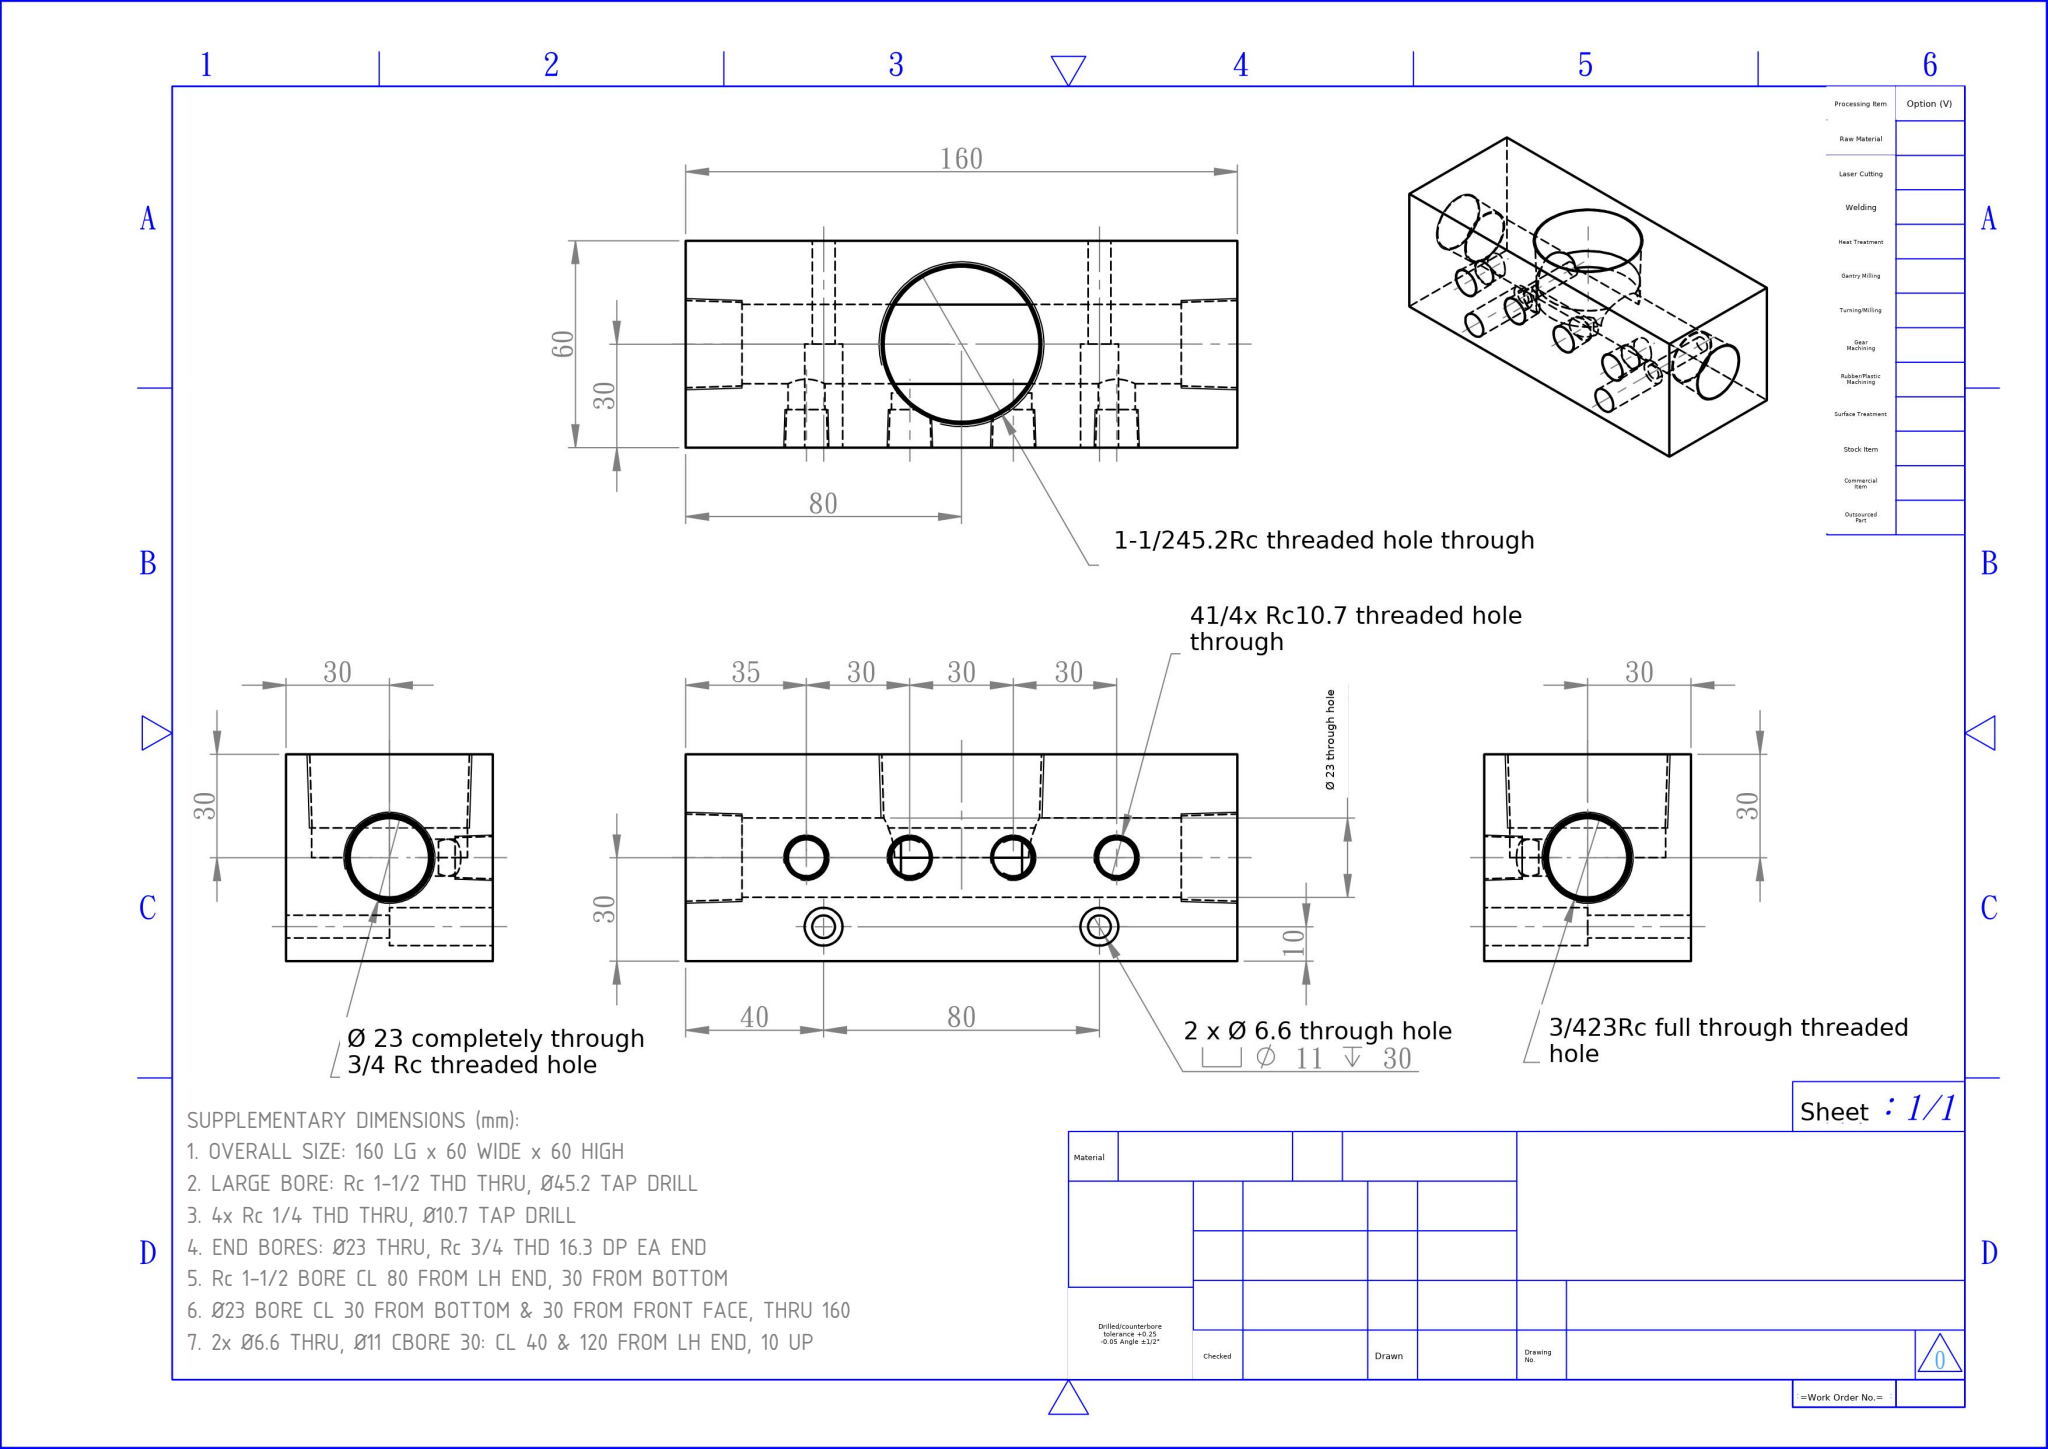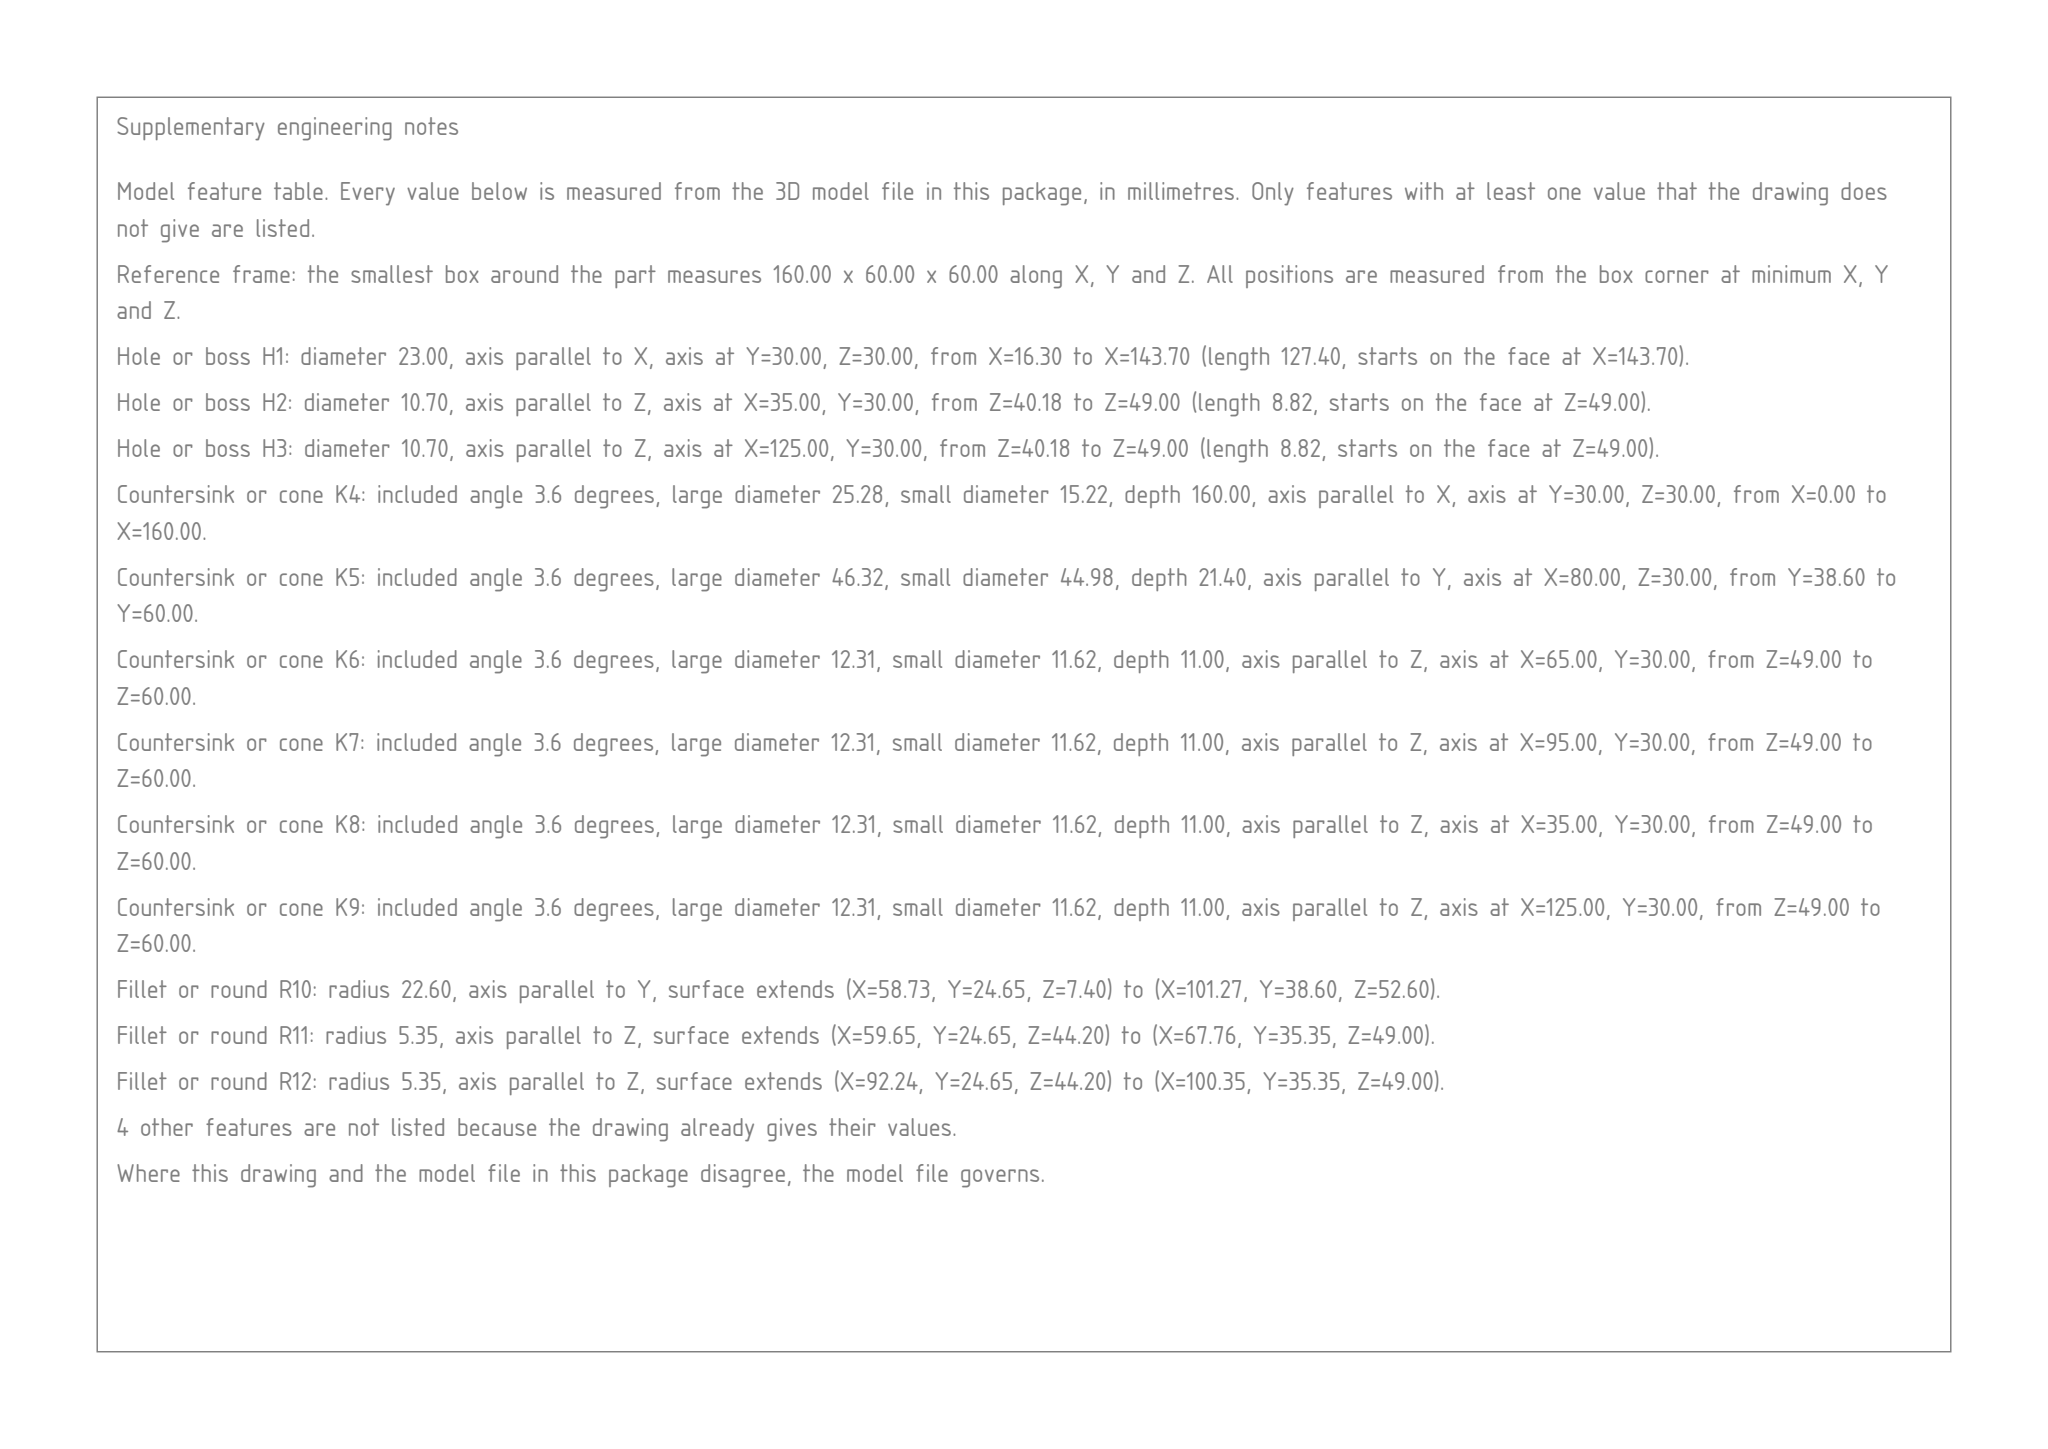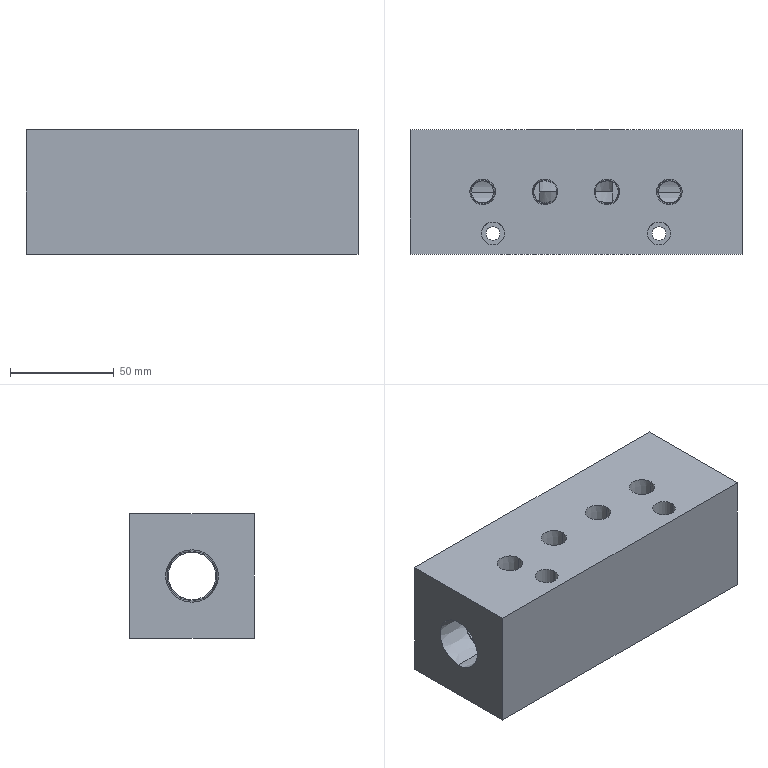Part | SolidWorks | mm | 1 solid | 57 faces | box 160 x 60 x 60 mm | volume 453102 mm3 | cylinder 23 | plane 20 | cone 14 | commonest cylinder face diameters 10.7 x7 45.2 x5 11 x4 6.6 x4 23 x3